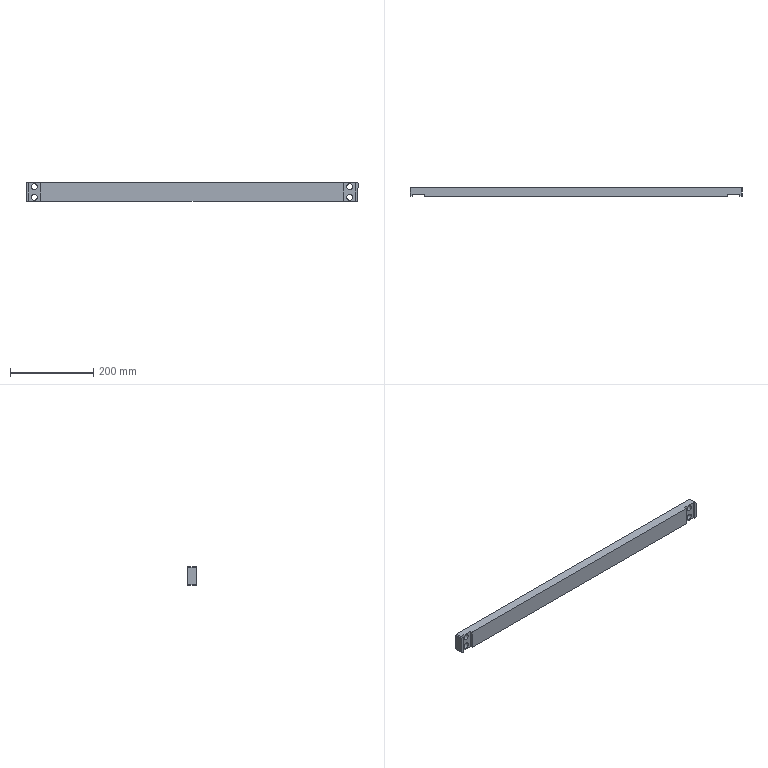Component | SolidWorks | FE5-217--p_O-1 | 1 solid | 26 faces | box 798 x 21 x 45 mm | volume 730590 mm3 | plane 18 | cylinder 8 | commonest cylinder face diameters 14 x8
build123d program:
from build123d import *

# Parameters (mm, degrees)
SKETCH1_W      = 798
SKETCH1_H      = 45
EXTRUDE1_DEPTH = 21
SKETCH2_W      = 30
SKETCH2_H      = 45
EXTRUDE2_DEPTH = 5
SKETCH3_R      = 7
EXTRUDE3_DEPTH = 401.185
CHAMFER1_SIZE  = 2


with BuildPart() as part:
    # Sketch1 → Extrude1 (new body)
    with BuildSketch(Plane(origin=(0, 0, 0), x_dir=(1, 0, 0), z_dir=(0, 1, 0))):
        Rectangle(SKETCH1_W, SKETCH1_H)
    extrude(amount=EXTRUDE1_DEPTH)

    # Sketch2 → Extrude2 (cut)
    with BuildSketch(Plane(origin=(0, 21, 0), x_dir=(1, 0, 0), z_dir=(0, 1, 0))):
        with Locations((379, 0)):
            Rectangle(SKETCH2_W, SKETCH2_H)
        with Locations((-379, 0)):
            Rectangle(SKETCH2_W, SKETCH2_H)
    extrude(amount=-EXTRUDE2_DEPTH, mode=Mode.SUBTRACT)

    # Sketch3 → Extrude3 (cut, through all)
    with BuildSketch(Plane(origin=(0, 21, 0), x_dir=(1, 0, 0), z_dir=(0, 1, 0))):
        with Locations(Location((379, 12.5, 0), (0, 0, 270))):
            Circle(SKETCH3_R)
        with Locations(Location((379, -12.5, 0), (0, 0, 270))):
            Circle(SKETCH3_R)
        with Locations(Location((-379, -12.5, 0), (0, 0, 270))):
            Circle(SKETCH3_R)
        with Locations(Location((-379, 12.5, 0), (0, 0, 270))):
            Circle(SKETCH3_R)
    extrude(amount=-EXTRUDE3_DEPTH, mode=Mode.SUBTRACT)

    # Chamfer1
    chamfer1_edges = [part.edges().sort_by_distance(p)[0] for p in [
        (-399, 10.5, -22.5),
        (399, 10.5, -22.5),
        (399, 10.5, 22.5),
        (-399, 10.5, 22.5),
    ]]
    chamfer(chamfer1_edges, length=CHAMFER1_SIZE)


solid = part.part

# Placed as in the assembly
solid = solid.moved(Location((-379, 125.5, -222.5), (180, 0, 0)))
STEP:
#1=CARTESIAN_POINT('',(-29.843,4.941,-7.992));
#2=VERTEX_POINT('',#1);
#3=CARTESIAN_POINT('',(-29.843,4.941,-8.543));
#4=VERTEX_POINT('',#3);
#5=CARTESIAN_POINT('',(-29.843,4.941,-8.268));
#6=DIRECTION('',(0.,-1.,0.));
#7=DIRECTION('',(0.,0.,1.));
#8=AXIS2_PLACEMENT_3D('',#5,#6,#7);
#9=CIRCLE('',#8,0.2756);
#10=EDGE_CURVE('',#2,#4,#9,.T.);
#11=ORIENTED_EDGE('',*,*,#10,.F.);
#12=CARTESIAN_POINT('',(-29.843,4.311,-7.992));
#13=VERTEX_POINT('',#12);
#14=CARTESIAN_POINT('',(-29.843,4.941,-7.992));
#15=DIRECTION('',(0.,-1.,0.));
#16=VECTOR('',#15,39.37);
#17=LINE('',#14,#16);
#18=EDGE_CURVE('',#2,#13,#17,.T.);
#19=ORIENTED_EDGE('',*,*,#18,.T.);
#20=CARTESIAN_POINT('',(-29.843,4.311,-8.543));
#21=VERTEX_POINT('',#20);
#22=CARTESIAN_POINT('',(-29.843,4.311,-8.268));
#23=DIRECTION('',(0.,-1.,0.));
#24=DIRECTION('',(0.,0.,-1.));
#25=AXIS2_PLACEMENT_3D('',#22,#23,#24);
#26=CIRCLE('',#25,0.2756);
#27=EDGE_CURVE('',#13,#21,#26,.T.);
#28=ORIENTED_EDGE('',*,*,#27,.T.);
#29=CARTESIAN_POINT('',(-29.843,4.941,-8.543));
#30=DIRECTION('',(0.,-1.,0.));
#31=VECTOR('',#30,39.37);
#32=LINE('',#29,#31);
#33=EDGE_CURVE('',#4,#21,#32,.T.);
#34=ORIENTED_EDGE('',*,*,#33,.F.);
#35=EDGE_LOOP('',(#11,#19,#28,#34));
#36=FACE_OUTER_BOUND('',#35,.T.);
#37=CARTESIAN_POINT('',(-29.843,4.941,-8.268));
#38=DIRECTION('',(0.,-1.,0.));
#39=DIRECTION('',(0.,0.,-1.));
#40=AXIS2_PLACEMENT_3D('',#37,#38,#39);
#41=CYLINDRICAL_SURFACE('',#40,0.2756);
#42=ADVANCED_FACE('',(#36),#41,.F.);
#43=CARTESIAN_POINT('',(-29.843,4.941,-8.976));
#44=VERTEX_POINT('',#43);
#45=CARTESIAN_POINT('',(-29.843,4.941,-9.528));
#46=VERTEX_POINT('',#45);
#47=CARTESIAN_POINT('',(-29.843,4.941,-9.252));
#48=DIRECTION('',(0.,-1.,0.));
#49=DIRECTION('',(0.,0.,-1.));
#50=AXIS2_PLACEMENT_3D('',#47,#48,#49);
#51=CIRCLE('',#50,0.2756);
#52=EDGE_CURVE('',#44,#46,#51,.T.);
#53=ORIENTED_EDGE('',*,*,#52,.F.);
#54=CARTESIAN_POINT('',(-29.843,4.311,-8.976));
#55=VERTEX_POINT('',#54);
#56=CARTESIAN_POINT('',(-29.843,4.941,-8.976));
#57=DIRECTION('',(0.,-1.,0.));
#58=VECTOR('',#57,39.37);
#59=LINE('',#56,#58);
#60=EDGE_CURVE('',#44,#55,#59,.T.);
#61=ORIENTED_EDGE('',*,*,#60,.T.);
#62=CARTESIAN_POINT('',(-29.843,4.311,-9.528));
#63=VERTEX_POINT('',#62);
#64=CARTESIAN_POINT('',(-29.843,4.311,-9.252));
#65=DIRECTION('',(0.,-1.,0.));
#66=DIRECTION('',(0.,0.,-1.));
#67=AXIS2_PLACEMENT_3D('',#64,#65,#66);
#68=CIRCLE('',#67,0.2756);
#69=EDGE_CURVE('',#55,#63,#68,.T.);
#70=ORIENTED_EDGE('',*,*,#69,.T.);
#71=CARTESIAN_POINT('',(-29.843,4.941,-9.528));
#72=DIRECTION('',(0.,-1.,0.));
#73=VECTOR('',#72,39.37);
#74=LINE('',#71,#73);
#75=EDGE_CURVE('',#46,#63,#74,.T.);
#76=ORIENTED_EDGE('',*,*,#75,.F.);
#77=EDGE_LOOP('',(#53,#61,#70,#76));
#78=FACE_OUTER_BOUND('',#77,.T.);
#79=CARTESIAN_POINT('',(-29.843,4.941,-9.252));
#80=DIRECTION('',(0.,-1.,0.));
#81=DIRECTION('',(0.,0.,-1.));
#82=AXIS2_PLACEMENT_3D('',#79,#80,#81);
#83=CYLINDRICAL_SURFACE('',#82,0.2756);
#84=ADVANCED_FACE('',(#78),#83,.F.);
#85=CARTESIAN_POINT('',(-0.,4.941,-8.976));
#86=VERTEX_POINT('',#85);
#87=CARTESIAN_POINT('',(-0.,4.941,-9.528));
#88=VERTEX_POINT('',#87);
#89=CARTESIAN_POINT('',(-0.,4.941,-9.252));
#90=DIRECTION('',(0.,-1.,0.));
#91=DIRECTION('',(0.,0.,1.));
#92=AXIS2_PLACEMENT_3D('',#89,#90,#91);
#93=CIRCLE('',#92,0.2756);
#94=EDGE_CURVE('',#86,#88,#93,.T.);
#95=ORIENTED_EDGE('',*,*,#94,.F.);
#96=CARTESIAN_POINT('',(-0.,4.311,-8.976));
#97=VERTEX_POINT('',#96);
#98=CARTESIAN_POINT('',(-0.,4.941,-8.976));
#99=DIRECTION('',(0.,-1.,0.));
#100=VECTOR('',#99,39.37);
#101=LINE('',#98,#100);
#102=EDGE_CURVE('',#86,#97,#101,.T.);
#103=ORIENTED_EDGE('',*,*,#102,.T.);
#104=CARTESIAN_POINT('',(-0.,4.311,-9.528));
#105=VERTEX_POINT('',#104);
#106=CARTESIAN_POINT('',(-0.,4.311,-9.252));
#107=DIRECTION('',(0.,-1.,0.));
#108=DIRECTION('',(-0.,0.,-1.));
#109=AXIS2_PLACEMENT_3D('',#106,#107,#108);
#110=CIRCLE('',#109,0.2756);
#111=EDGE_CURVE('',#97,#105,#110,.T.);
#112=ORIENTED_EDGE('',*,*,#111,.T.);
#113=CARTESIAN_POINT('',(-0.,4.941,-9.528));
#114=DIRECTION('',(0.,-1.,0.));
#115=VECTOR('',#114,39.37);
#116=LINE('',#113,#115);
#117=EDGE_CURVE('',#88,#105,#116,.T.);
#118=ORIENTED_EDGE('',*,*,#117,.F.);
#119=EDGE_LOOP('',(#95,#103,#112,#118));
#120=FACE_OUTER_BOUND('',#119,.T.);
#121=CARTESIAN_POINT('',(-0.,4.941,-9.252));
#122=DIRECTION('',(0.,-1.,0.));
#123=DIRECTION('',(-0.,0.,-1.));
#124=AXIS2_PLACEMENT_3D('',#121,#122,#123);
#125=CYLINDRICAL_SURFACE('',#124,0.2756);
#126=ADVANCED_FACE('',(#120),#125,.F.);
#127=CARTESIAN_POINT('',(-0.,4.941,-7.992));
#128=VERTEX_POINT('',#127);
#129=CARTESIAN_POINT('',(-0.,4.941,-8.543));
#130=VERTEX_POINT('',#129);
#131=CARTESIAN_POINT('',(-0.,4.941,-8.268));
#132=DIRECTION('',(0.,-1.,0.));
#133=DIRECTION('',(-0.,0.,-1.));
#134=AXIS2_PLACEMENT_3D('',#131,#132,#133);
#135=CIRCLE('',#134,0.2756);
#136=EDGE_CURVE('',#128,#130,#135,.T.);
#137=ORIENTED_EDGE('',*,*,#136,.F.);
#138=CARTESIAN_POINT('',(-0.,4.311,-7.992));
#139=VERTEX_POINT('',#138);
#140=CARTESIAN_POINT('',(-0.,4.941,-7.992));
#141=DIRECTION('',(0.,-1.,0.));
#142=VECTOR('',#141,39.37);
#143=LINE('',#140,#142);
#144=EDGE_CURVE('',#128,#139,#143,.T.);
#145=ORIENTED_EDGE('',*,*,#144,.T.);
#146=CARTESIAN_POINT('',(-0.,4.311,-8.543));
#147=VERTEX_POINT('',#146);
#148=CARTESIAN_POINT('',(-0.,4.311,-8.268));
#149=DIRECTION('',(0.,-1.,0.));
#150=DIRECTION('',(-0.,0.,-1.));
#151=AXIS2_PLACEMENT_3D('',#148,#149,#150);
#152=CIRCLE('',#151,0.2756);
#153=EDGE_CURVE('',#139,#147,#152,.T.);
#154=ORIENTED_EDGE('',*,*,#153,.T.);
#155=CARTESIAN_POINT('',(-0.,4.941,-8.543));
#156=DIRECTION('',(0.,-1.,0.));
#157=VECTOR('',#156,39.37);
#158=LINE('',#155,#157);
#159=EDGE_CURVE('',#130,#147,#158,.T.);
#160=ORIENTED_EDGE('',*,*,#159,.F.);
#161=EDGE_LOOP('',(#137,#145,#154,#160));
#162=FACE_OUTER_BOUND('',#161,.T.);
#163=CARTESIAN_POINT('',(-0.,4.941,-8.268));
#164=DIRECTION('',(0.,-1.,0.));
#165=DIRECTION('',(-0.,0.,-1.));
#166=AXIS2_PLACEMENT_3D('',#163,#164,#165);
#167=CYLINDRICAL_SURFACE('',#166,0.2756);
#168=ADVANCED_FACE('',(#162),#167,.F.);
#169=CARTESIAN_POINT('',(-29.252,4.114,-9.646));
#170=VERTEX_POINT('',#169);
#171=CARTESIAN_POINT('',(-29.252,4.114,-7.874));
#172=VERTEX_POINT('',#171);
#173=CARTESIAN_POINT('',(-29.252,4.114,-7.874));
#174=DIRECTION('',(0.,0.,1.));
#175=VECTOR('',#174,39.37);
#176=LINE('',#173,#175);
#177=EDGE_CURVE('',#170,#172,#176,.T.);
#178=ORIENTED_EDGE('',*,*,#177,.F.);
#179=CARTESIAN_POINT('',(-0.5906,4.114,-9.646));
#180=VERTEX_POINT('',#179);
#181=CARTESIAN_POINT('',(0.7874,4.114,-9.646));
#182=DIRECTION('',(1.,0.,-0.));
#183=VECTOR('',#182,39.37);
#184=LINE('',#181,#183);
#185=EDGE_CURVE('',#170,#180,#184,.T.);
#186=ORIENTED_EDGE('',*,*,#185,.T.);
#187=CARTESIAN_POINT('',(-0.5906,4.114,-7.874));
#188=VERTEX_POINT('',#187);
#189=CARTESIAN_POINT('',(-0.5906,4.114,-7.874));
#190=DIRECTION('',(-0.,0.,-1.));
#191=VECTOR('',#190,39.37);
#192=LINE('',#189,#191);
#193=EDGE_CURVE('',#188,#180,#192,.T.);
#194=ORIENTED_EDGE('',*,*,#193,.F.);
#195=CARTESIAN_POINT('',(0.7874,4.114,-7.874));
#196=DIRECTION('',(-1.,0.,0.));
#197=VECTOR('',#196,39.37);
#198=LINE('',#195,#197);
#199=EDGE_CURVE('',#188,#172,#198,.T.);
#200=ORIENTED_EDGE('',*,*,#199,.T.);
#201=EDGE_LOOP('',(#178,#186,#194,#200));
#202=FACE_OUTER_BOUND('',#201,.T.);
#203=CARTESIAN_POINT('',(-30.63,4.114,-7.874));
#204=DIRECTION('',(0.,-1.,0.));
#205=DIRECTION('',(-0.,0.,-1.));
#206=AXIS2_PLACEMENT_3D('',#203,#204,#205);
#207=PLANE('',#206);
#208=ADVANCED_FACE('',(#202),#207,.T.);
#209=CARTESIAN_POINT('',(-30.433,4.114,-7.874));
#210=VERTEX_POINT('',#209);
#211=CARTESIAN_POINT('',(-30.551,4.114,-7.874));
#212=VERTEX_POINT('',#211);
#213=CARTESIAN_POINT('',(0.7874,4.114,-7.874));
#214=DIRECTION('',(-1.,0.,0.));
#215=VECTOR('',#214,39.37);
#216=LINE('',#213,#215);
#217=EDGE_CURVE('',#210,#212,#216,.T.);
#218=ORIENTED_EDGE('',*,*,#217,.T.);
#219=CARTESIAN_POINT('',(-30.63,4.114,-7.953));
#220=VERTEX_POINT('',#219);
#221=CARTESIAN_POINT('',(-30.591,4.114,-7.913));
#222=DIRECTION('',(-0.7071,0.,-0.7071));
#223=VECTOR('',#222,39.37);
#224=LINE('',#221,#223);
#225=EDGE_CURVE('',#212,#220,#224,.T.);
#226=ORIENTED_EDGE('',*,*,#225,.T.);
#227=CARTESIAN_POINT('',(-30.63,4.114,-9.567));
#228=VERTEX_POINT('',#227);
#229=CARTESIAN_POINT('',(-30.63,4.114,-9.646));
#230=DIRECTION('',(-0.,0.,-1.));
#231=VECTOR('',#230,39.37);
#232=LINE('',#229,#231);
#233=EDGE_CURVE('',#220,#228,#232,.T.);
#234=ORIENTED_EDGE('',*,*,#233,.T.);
#235=CARTESIAN_POINT('',(-30.551,4.114,-9.646));
#236=VERTEX_POINT('',#235);
#237=CARTESIAN_POINT('',(-31.476,4.114,-8.72));
#238=DIRECTION('',(0.7071,0.,-0.7071));
#239=VECTOR('',#238,39.37);
#240=LINE('',#237,#239);
#241=EDGE_CURVE('',#228,#236,#240,.T.);
#242=ORIENTED_EDGE('',*,*,#241,.T.);
#243=CARTESIAN_POINT('',(-30.433,4.114,-9.646));
#244=VERTEX_POINT('',#243);
#245=CARTESIAN_POINT('',(0.7874,4.114,-9.646));
#246=DIRECTION('',(1.,0.,-0.));
#247=VECTOR('',#246,39.37);
#248=LINE('',#245,#247);
#249=EDGE_CURVE('',#236,#244,#248,.T.);
#250=ORIENTED_EDGE('',*,*,#249,.T.);
#251=CARTESIAN_POINT('',(-30.433,4.114,-7.874));
#252=DIRECTION('',(-0.,0.,-1.));
#253=VECTOR('',#252,39.37);
#254=LINE('',#251,#253);
#255=EDGE_CURVE('',#210,#244,#254,.T.);
#256=ORIENTED_EDGE('',*,*,#255,.F.);
#257=EDGE_LOOP('',(#218,#226,#234,#242,#250,#256));
#258=FACE_OUTER_BOUND('',#257,.T.);
#259=CARTESIAN_POINT('',(-30.63,4.114,-7.874));
#260=DIRECTION('',(0.,-1.,0.));
#261=DIRECTION('',(-0.,0.,-1.));
#262=AXIS2_PLACEMENT_3D('',#259,#260,#261);
#263=PLANE('',#262);
#264=ADVANCED_FACE('',(#258),#263,.T.);
#265=ORIENTED_EDGE('',*,*,#233,.F.);
#266=CARTESIAN_POINT('',(-30.63,4.941,-7.953));
#267=VERTEX_POINT('',#266);
#268=CARTESIAN_POINT('',(-30.63,4.114,-7.953));
#269=DIRECTION('',(0.,1.,0.));
#270=VECTOR('',#269,39.37);
#271=LINE('',#268,#270);
#272=EDGE_CURVE('',#220,#267,#271,.T.);
#273=ORIENTED_EDGE('',*,*,#272,.T.);
#274=CARTESIAN_POINT('',(-30.63,4.941,-9.567));
#275=VERTEX_POINT('',#274);
#276=CARTESIAN_POINT('',(-30.63,4.941,-9.646));
#277=DIRECTION('',(-0.,0.,-1.));
#278=VECTOR('',#277,39.37);
#279=LINE('',#276,#278);
#280=EDGE_CURVE('',#267,#275,#279,.T.);
#281=ORIENTED_EDGE('',*,*,#280,.T.);
#282=CARTESIAN_POINT('',(-30.63,4.114,-9.567));
#283=DIRECTION('',(0.,-1.,0.));
#284=VECTOR('',#283,39.37);
#285=LINE('',#282,#284);
#286=EDGE_CURVE('',#275,#228,#285,.T.);
#287=ORIENTED_EDGE('',*,*,#286,.T.);
#288=EDGE_LOOP('',(#265,#273,#281,#287));
#289=FACE_OUTER_BOUND('',#288,.T.);
#290=CARTESIAN_POINT('',(-30.63,4.114,-9.646));
#291=DIRECTION('',(1.,0.,-0.));
#292=DIRECTION('',(0.,0.,1.));
#293=AXIS2_PLACEMENT_3D('',#290,#291,#292);
#294=PLANE('',#293);
#295=ADVANCED_FACE('',(#289),#294,.F.);
#296=ORIENTED_EDGE('',*,*,#249,.F.);
#297=CARTESIAN_POINT('',(-30.551,4.941,-9.646));
#298=VERTEX_POINT('',#297);
#299=CARTESIAN_POINT('',(-30.551,4.114,-9.646));
#300=DIRECTION('',(0.,1.,0.));
#301=VECTOR('',#300,39.37);
#302=LINE('',#299,#301);
#303=EDGE_CURVE('',#236,#298,#302,.T.);
#304=ORIENTED_EDGE('',*,*,#303,.T.);
#305=CARTESIAN_POINT('',(0.7087,4.941,-9.646));
#306=VERTEX_POINT('',#305);
#307=CARTESIAN_POINT('',(0.7874,4.941,-9.646));
#308=DIRECTION('',(1.,0.,-0.));
#309=VECTOR('',#308,39.37);
#310=LINE('',#307,#309);
#311=EDGE_CURVE('',#298,#306,#310,.T.);
#312=ORIENTED_EDGE('',*,*,#311,.T.);
#313=CARTESIAN_POINT('',(0.7087,4.114,-9.646));
#314=VERTEX_POINT('',#313);
#315=CARTESIAN_POINT('',(0.7087,4.114,-9.646));
#316=DIRECTION('',(0.,-1.,0.));
#317=VECTOR('',#316,39.37);
#318=LINE('',#315,#317);
#319=EDGE_CURVE('',#306,#314,#318,.T.);
#320=ORIENTED_EDGE('',*,*,#319,.T.);
#321=CARTESIAN_POINT('',(0.5906,4.114,-9.646));
#322=VERTEX_POINT('',#321);
#323=CARTESIAN_POINT('',(0.7874,4.114,-9.646));
#324=DIRECTION('',(1.,0.,-0.));
#325=VECTOR('',#324,39.37);
#326=LINE('',#323,#325);
#327=EDGE_CURVE('',#322,#314,#326,.T.);
#328=ORIENTED_EDGE('',*,*,#327,.F.);
#329=CARTESIAN_POINT('',(0.5906,4.311,-9.646));
#330=VERTEX_POINT('',#329);
#331=CARTESIAN_POINT('',(0.5906,4.311,-9.646));
#332=DIRECTION('',(0.,-1.,0.));
#333=VECTOR('',#332,39.37);
#334=LINE('',#331,#333);
#335=EDGE_CURVE('',#330,#322,#334,.T.);
#336=ORIENTED_EDGE('',*,*,#335,.F.);
#337=CARTESIAN_POINT('',(-0.5906,4.311,-9.646));
#338=VERTEX_POINT('',#337);
#339=CARTESIAN_POINT('',(-0.5906,4.311,-9.646));
#340=DIRECTION('',(1.,0.,-0.));
#341=VECTOR('',#340,39.37);
#342=LINE('',#339,#341);
#343=EDGE_CURVE('',#338,#330,#342,.T.);
#344=ORIENTED_EDGE('',*,*,#343,.F.);
#345=CARTESIAN_POINT('',(-0.5906,4.311,-9.646));
#346=DIRECTION('',(0.,-1.,0.));
#347=VECTOR('',#346,39.37);
#348=LINE('',#345,#347);
#349=EDGE_CURVE('',#338,#180,#348,.T.);
#350=ORIENTED_EDGE('',*,*,#349,.T.);
#351=ORIENTED_EDGE('',*,*,#185,.F.);
#352=CARTESIAN_POINT('',(-29.252,4.311,-9.646));
#353=VERTEX_POINT('',#352);
#354=CARTESIAN_POINT('',(-29.252,4.311,-9.646));
#355=DIRECTION('',(0.,-1.,0.));
#356=VECTOR('',#355,39.37);
#357=LINE('',#354,#356);
#358=EDGE_CURVE('',#353,#170,#357,.T.);
#359=ORIENTED_EDGE('',*,*,#358,.F.);
#360=CARTESIAN_POINT('',(-30.433,4.311,-9.646));
#361=VERTEX_POINT('',#360);
#362=CARTESIAN_POINT('',(-29.252,4.311,-9.646));
#363=DIRECTION('',(1.,0.,-0.));
#364=VECTOR('',#363,39.37);
#365=LINE('',#362,#364);
#366=EDGE_CURVE('',#361,#353,#365,.T.);
#367=ORIENTED_EDGE('',*,*,#366,.F.);
#368=CARTESIAN_POINT('',(-30.433,4.311,-9.646));
#369=DIRECTION('',(0.,-1.,0.));
#370=VECTOR('',#369,39.37);
#371=LINE('',#368,#370);
#372=EDGE_CURVE('',#361,#244,#371,.T.);
#373=ORIENTED_EDGE('',*,*,#372,.T.);
#374=EDGE_LOOP('',(#296,#304,#312,#320,#328,#336,#344,#350,#351,#359,#367,#373));
#375=FACE_OUTER_BOUND('',#374,.T.);
#376=CARTESIAN_POINT('',(0.7874,4.114,-9.646));
#377=DIRECTION('',(0.,0.,1.));
#378=DIRECTION('',(-1.,0.,0.));
#379=AXIS2_PLACEMENT_3D('',#376,#377,#378);
#380=PLANE('',#379);
#381=ADVANCED_FACE('',(#375),#380,.F.);
#382=CARTESIAN_POINT('',(0.7874,4.941,-9.567));
#383=VERTEX_POINT('',#382);
#384=CARTESIAN_POINT('',(0.7874,4.941,-7.953));
#385=VERTEX_POINT('',#384);
#386=CARTESIAN_POINT('',(0.7874,4.941,-9.646));
#387=DIRECTION('',(0.,0.,1.));
#388=VECTOR('',#387,39.37);
#389=LINE('',#386,#388);
#390=EDGE_CURVE('',#383,#385,#389,.T.);
#391=ORIENTED_EDGE('',*,*,#390,.T.);
#392=CARTESIAN_POINT('',(0.7874,4.114,-7.953));
#393=VERTEX_POINT('',#392);
#394=CARTESIAN_POINT('',(0.7874,4.114,-7.953));
#395=DIRECTION('',(0.,-1.,0.));
#396=VECTOR('',#395,39.37);
#397=LINE('',#394,#396);
#398=EDGE_CURVE('',#385,#393,#397,.T.);
#399=ORIENTED_EDGE('',*,*,#398,.T.);
#400=CARTESIAN_POINT('',(0.7874,4.114,-9.567));
#401=VERTEX_POINT('',#400);
#402=CARTESIAN_POINT('',(0.7874,4.114,-9.646));
#403=DIRECTION('',(0.,0.,1.));
#404=VECTOR('',#403,39.37);
#405=LINE('',#402,#404);
#406=EDGE_CURVE('',#401,#393,#405,.T.);
#407=ORIENTED_EDGE('',*,*,#406,.F.);
#408=CARTESIAN_POINT('',(0.7874,4.114,-9.567));
#409=DIRECTION('',(0.,1.,0.));
#410=VECTOR('',#409,39.37);
#411=LINE('',#408,#410);
#412=EDGE_CURVE('',#401,#383,#411,.T.);
#413=ORIENTED_EDGE('',*,*,#412,.T.);
#414=EDGE_LOOP('',(#391,#399,#407,#413));
#415=FACE_OUTER_BOUND('',#414,.T.);
#416=CARTESIAN_POINT('',(0.7874,4.114,-9.646));
#417=DIRECTION('',(-1.,0.,0.));
#418=DIRECTION('',(-0.,0.,-1.));
#419=AXIS2_PLACEMENT_3D('',#416,#417,#418);
#420=PLANE('',#419);
#421=ADVANCED_FACE('',(#415),#420,.F.);
#422=CARTESIAN_POINT('',(0.7087,4.941,-7.874));
#423=VERTEX_POINT('',#422);
#424=CARTESIAN_POINT('',(-30.551,4.941,-7.874));
#425=VERTEX_POINT('',#424);
#426=CARTESIAN_POINT('',(0.7874,4.941,-7.874));
#427=DIRECTION('',(-1.,0.,0.));
#428=VECTOR('',#427,39.37);
#429=LINE('',#426,#428);
#430=EDGE_CURVE('',#423,#425,#429,.T.);
#431=ORIENTED_EDGE('',*,*,#430,.T.);
#432=CARTESIAN_POINT('',(-30.551,4.114,-7.874));
#433=DIRECTION('',(0.,-1.,0.));
#434=VECTOR('',#433,39.37);
#435=LINE('',#432,#434);
#436=EDGE_CURVE('',#425,#212,#435,.T.);
#437=ORIENTED_EDGE('',*,*,#436,.T.);
#438=ORIENTED_EDGE('',*,*,#217,.F.);
#439=CARTESIAN_POINT('',(-30.433,4.311,-7.874));
#440=VERTEX_POINT('',#439);
#441=CARTESIAN_POINT('',(-30.433,4.311,-7.874));
#442=DIRECTION('',(0.,-1.,0.));
#443=VECTOR('',#442,39.37);
#444=LINE('',#441,#443);
#445=EDGE_CURVE('',#440,#210,#444,.T.);
#446=ORIENTED_EDGE('',*,*,#445,.F.);
#447=CARTESIAN_POINT('',(-29.252,4.311,-7.874));
#448=VERTEX_POINT('',#447);
#449=CARTESIAN_POINT('',(-29.252,4.311,-7.874));
#450=DIRECTION('',(-1.,0.,0.));
#451=VECTOR('',#450,39.37);
#452=LINE('',#449,#451);
#453=EDGE_CURVE('',#448,#440,#452,.T.);
#454=ORIENTED_EDGE('',*,*,#453,.F.);
#455=CARTESIAN_POINT('',(-29.252,4.311,-7.874));
#456=DIRECTION('',(0.,-1.,0.));
#457=VECTOR('',#456,39.37);
#458=LINE('',#455,#457);
#459=EDGE_CURVE('',#448,#172,#458,.T.);
#460=ORIENTED_EDGE('',*,*,#459,.T.);
#461=ORIENTED_EDGE('',*,*,#199,.F.);
#462=CARTESIAN_POINT('',(-0.5906,4.311,-7.874));
#463=VERTEX_POINT('',#462);
#464=CARTESIAN_POINT('',(-0.5906,4.311,-7.874));
#465=DIRECTION('',(0.,-1.,0.));
#466=VECTOR('',#465,39.37);
#467=LINE('',#464,#466);
#468=EDGE_CURVE('',#463,#188,#467,.T.);
#469=ORIENTED_EDGE('',*,*,#468,.F.);
#470=CARTESIAN_POINT('',(0.5906,4.311,-7.874));
#471=VERTEX_POINT('',#470);
#472=CARTESIAN_POINT('',(-0.5906,4.311,-7.874));
#473=DIRECTION('',(-1.,0.,0.));
#474=VECTOR('',#473,39.37);
#475=LINE('',#472,#474);
#476=EDGE_CURVE('',#471,#463,#475,.T.);
#477=ORIENTED_EDGE('',*,*,#476,.F.);
#478=CARTESIAN_POINT('',(0.5906,4.114,-7.874));
#479=VERTEX_POINT('',#478);
#480=CARTESIAN_POINT('',(0.5906,4.311,-7.874));
#481=DIRECTION('',(0.,-1.,0.));
#482=VECTOR('',#481,39.37);
#483=LINE('',#480,#482);
#484=EDGE_CURVE('',#471,#479,#483,.T.);
#485=ORIENTED_EDGE('',*,*,#484,.T.);
#486=CARTESIAN_POINT('',(0.7087,4.114,-7.874));
#487=VERTEX_POINT('',#486);
#488=CARTESIAN_POINT('',(0.7874,4.114,-7.874));
#489=DIRECTION('',(-1.,0.,0.));
#490=VECTOR('',#489,39.37);
#491=LINE('',#488,#490);
#492=EDGE_CURVE('',#487,#479,#491,.T.);
#493=ORIENTED_EDGE('',*,*,#492,.F.);
#494=CARTESIAN_POINT('',(0.7087,4.114,-7.874));
#495=DIRECTION('',(0.,1.,0.));
#496=VECTOR('',#495,39.37);
#497=LINE('',#494,#496);
#498=EDGE_CURVE('',#487,#423,#497,.T.);
#499=ORIENTED_EDGE('',*,*,#498,.T.);
#500=EDGE_LOOP('',(#431,#437,#438,#446,#454,#460,#461,#469,#477,#485,#493,#499));
#501=FACE_OUTER_BOUND('',#500,.T.);
#502=CARTESIAN_POINT('',(0.7874,4.114,-7.874));
#503=DIRECTION('',(-0.,0.,-1.));
#504=DIRECTION('',(1.,0.,-0.));
#505=AXIS2_PLACEMENT_3D('',#502,#503,#504);
#506=PLANE('',#505);
#507=ADVANCED_FACE('',(#501),#506,.F.);
#508=ORIENTED_EDGE('',*,*,#406,.T.);
#509=CARTESIAN_POINT('',(-14.961,4.114,7.795));
#510=DIRECTION('',(-0.7071,0.,0.7071));
#511=VECTOR('',#510,39.37);
#512=LINE('',#509,#511);
#513=EDGE_CURVE('',#393,#487,#512,.T.);
#514=ORIENTED_EDGE('',*,*,#513,.T.);
#515=ORIENTED_EDGE('',*,*,#492,.T.);
#516=CARTESIAN_POINT('',(0.5906,4.114,-7.874));
#517=DIRECTION('',(0.,0.,1.));
#518=VECTOR('',#517,39.37);
#519=LINE('',#516,#518);
#520=EDGE_CURVE('',#322,#479,#519,.T.);
#521=ORIENTED_EDGE('',*,*,#520,.F.);
#522=ORIENTED_EDGE('',*,*,#327,.T.);
#523=CARTESIAN_POINT('',(-14.075,4.114,-24.429));
#524=DIRECTION('',(0.7071,0.,0.7071));
#525=VECTOR('',#524,39.37);
#526=LINE('',#523,#525);
#527=EDGE_CURVE('',#314,#401,#526,.T.);
#528=ORIENTED_EDGE('',*,*,#527,.T.);
#529=EDGE_LOOP('',(#508,#514,#515,#521,#522,#528));
#530=FACE_OUTER_BOUND('',#529,.T.);
#531=CARTESIAN_POINT('',(-30.63,4.114,-7.874));
#532=DIRECTION('',(0.,-1.,0.));
#533=DIRECTION('',(-0.,0.,-1.));
#534=AXIS2_PLACEMENT_3D('',#531,#532,#533);
#535=PLANE('',#534);
#536=ADVANCED_FACE('',(#530),#535,.T.);
#537=CARTESIAN_POINT('',(-29.843,4.941,-8.268));
#538=DIRECTION('',(0.,-1.,0.));
#539=DIRECTION('',(0.,0.,1.));
#540=AXIS2_PLACEMENT_3D('',#537,#538,#539);
#541=CIRCLE('',#540,0.2756);
#542=EDGE_CURVE('',#4,#2,#541,.T.);
#543=ORIENTED_EDGE('',*,*,#542,.T.);
#544=ORIENTED_EDGE('',*,*,#10,.T.);
#545=EDGE_LOOP('',(#543,#544));
#546=FACE_BOUND('',#545,.T.);
#547=CARTESIAN_POINT('',(-29.843,4.941,-9.252));
#548=DIRECTION('',(0.,-1.,0.));
#549=DIRECTION('',(0.,0.,-1.));
#550=AXIS2_PLACEMENT_3D('',#547,#548,#549);
#551=CIRCLE('',#550,0.2756);
#552=EDGE_CURVE('',#46,#44,#551,.T.);
#553=ORIENTED_EDGE('',*,*,#552,.T.);
#554=ORIENTED_EDGE('',*,*,#52,.T.);
#555=EDGE_LOOP('',(#553,#554));
#556=FACE_BOUND('',#555,.T.);
#557=CARTESIAN_POINT('',(-0.,4.941,-9.252));
#558=DIRECTION('',(0.,-1.,0.));
#559=DIRECTION('',(0.,0.,1.));
#560=AXIS2_PLACEMENT_3D('',#557,#558,#559);
#561=CIRCLE('',#560,0.2756);
#562=EDGE_CURVE('',#88,#86,#561,.T.);
#563=ORIENTED_EDGE('',*,*,#562,.T.);
#564=ORIENTED_EDGE('',*,*,#94,.T.);
#565=EDGE_LOOP('',(#563,#564));
#566=FACE_BOUND('',#565,.T.);
#567=CARTESIAN_POINT('',(-0.,4.941,-8.268));
#568=DIRECTION('',(0.,-1.,0.));
#569=DIRECTION('',(-0.,0.,-1.));
#570=AXIS2_PLACEMENT_3D('',#567,#568,#569);
#571=CIRCLE('',#570,0.2756);
#572=EDGE_CURVE('',#130,#128,#571,.T.);
#573=ORIENTED_EDGE('',*,*,#572,.T.);
#574=ORIENTED_EDGE('',*,*,#136,.T.);
#575=EDGE_LOOP('',(#573,#574));
#576=FACE_BOUND('',#575,.T.);
#577=ORIENTED_EDGE('',*,*,#280,.F.);
#578=CARTESIAN_POINT('',(-30.63,4.941,-7.953));
#579=DIRECTION('',(0.7071,0.,0.7071));
#580=VECTOR('',#579,39.37);
#581=LINE('',#578,#580);
#582=EDGE_CURVE('',#267,#425,#581,.T.);
#583=ORIENTED_EDGE('',*,*,#582,.T.);
#584=ORIENTED_EDGE('',*,*,#430,.F.);
#585=CARTESIAN_POINT('',(0.7087,4.941,-7.874));
#586=DIRECTION('',(0.7071,0.,-0.7071));
#587=VECTOR('',#586,39.37);
#588=LINE('',#585,#587);
#589=EDGE_CURVE('',#423,#385,#588,.T.);
#590=ORIENTED_EDGE('',*,*,#589,.T.);
#591=ORIENTED_EDGE('',*,*,#390,.F.);
#592=CARTESIAN_POINT('',(0.7874,4.941,-9.567));
#593=DIRECTION('',(-0.7071,0.,-0.7071));
#594=VECTOR('',#593,39.37);
#595=LINE('',#592,#594);
#596=EDGE_CURVE('',#383,#306,#595,.T.);
#597=ORIENTED_EDGE('',*,*,#596,.T.);
#598=ORIENTED_EDGE('',*,*,#311,.F.);
#599=CARTESIAN_POINT('',(-30.551,4.941,-9.646));
#600=DIRECTION('',(-0.7071,0.,0.7071));
#601=VECTOR('',#600,39.37);
#602=LINE('',#599,#601);
#603=EDGE_CURVE('',#298,#275,#602,.T.);
#604=ORIENTED_EDGE('',*,*,#603,.T.);
#605=EDGE_LOOP('',(#577,#583,#584,#590,#591,#597,#598,#604));
#606=FACE_OUTER_BOUND('',#605,.T.);
#607=CARTESIAN_POINT('',(-30.63,4.941,-7.874));
#608=DIRECTION('',(0.,-1.,0.));
#609=DIRECTION('',(-0.,0.,-1.));
#610=AXIS2_PLACEMENT_3D('',#607,#608,#609);
#611=PLANE('',#610);
#612=ADVANCED_FACE('',(#546,#556,#566,#576,#606),#611,.F.);
#613=ORIENTED_EDGE('',*,*,#193,.T.);
#614=ORIENTED_EDGE('',*,*,#349,.F.);
#615=CARTESIAN_POINT('',(-0.5906,4.311,-7.874));
#616=DIRECTION('',(-0.,0.,-1.));
#617=VECTOR('',#616,39.37);
#618=LINE('',#615,#617);
#619=EDGE_CURVE('',#463,#338,#618,.T.);
#620=ORIENTED_EDGE('',*,*,#619,.F.);
#621=ORIENTED_EDGE('',*,*,#468,.T.);
#622=EDGE_LOOP('',(#613,#614,#620,#621));
#623=FACE_OUTER_BOUND('',#622,.T.);
#624=CARTESIAN_POINT('',(-0.5906,4.311,-7.874));
#625=DIRECTION('',(-1.,0.,0.));
#626=DIRECTION('',(-0.,0.,-1.));
#627=AXIS2_PLACEMENT_3D('',#624,#625,#626);
#628=PLANE('',#627);
#629=ADVANCED_FACE('',(#623),#628,.F.);
#630=ORIENTED_EDGE('',*,*,#520,.T.);
#631=ORIENTED_EDGE('',*,*,#484,.F.);
#632=CARTESIAN_POINT('',(0.5906,4.311,-7.874));
#633=DIRECTION('',(0.,0.,1.));
#634=VECTOR('',#633,39.37);
#635=LINE('',#632,#634);
#636=EDGE_CURVE('',#330,#471,#635,.T.);
#637=ORIENTED_EDGE('',*,*,#636,.F.);
#638=ORIENTED_EDGE('',*,*,#335,.T.);
#639=EDGE_LOOP('',(#630,#631,#637,#638));
#640=FACE_OUTER_BOUND('',#639,.T.);
#641=CARTESIAN_POINT('',(0.5906,4.311,-7.874));
#642=DIRECTION('',(1.,0.,-0.));
#643=DIRECTION('',(0.,0.,1.));
#644=AXIS2_PLACEMENT_3D('',#641,#642,#643);
#645=PLANE('',#644);
#646=ADVANCED_FACE('',(#640),#645,.F.);
#647=CARTESIAN_POINT('',(-0.,4.311,-9.252));
#648=DIRECTION('',(0.,-1.,0.));
#649=DIRECTION('',(-0.,0.,-1.));
#650=AXIS2_PLACEMENT_3D('',#647,#648,#649);
#651=CIRCLE('',#650,0.2756);
#652=EDGE_CURVE('',#105,#97,#651,.T.);
#653=ORIENTED_EDGE('',*,*,#652,.F.);
#654=ORIENTED_EDGE('',*,*,#111,.F.);
#655=EDGE_LOOP('',(#653,#654));
#656=FACE_BOUND('',#655,.T.);
#657=CARTESIAN_POINT('',(-0.,4.311,-8.268));
#658=DIRECTION('',(0.,-1.,0.));
#659=DIRECTION('',(-0.,0.,-1.));
#660=AXIS2_PLACEMENT_3D('',#657,#658,#659);
#661=CIRCLE('',#660,0.2756);
#662=EDGE_CURVE('',#147,#139,#661,.T.);
#663=ORIENTED_EDGE('',*,*,#662,.F.);
#664=ORIENTED_EDGE('',*,*,#153,.F.);
#665=EDGE_LOOP('',(#663,#664));
#666=FACE_BOUND('',#665,.T.);
#667=ORIENTED_EDGE('',*,*,#619,.T.);
#668=ORIENTED_EDGE('',*,*,#343,.T.);
#669=ORIENTED_EDGE('',*,*,#636,.T.);
#670=ORIENTED_EDGE('',*,*,#476,.T.);
#671=EDGE_LOOP('',(#667,#668,#669,#670));
#672=FACE_OUTER_BOUND('',#671,.T.);
#673=CARTESIAN_POINT('',(-0.5906,4.311,-9.646));
#674=DIRECTION('',(0.,-1.,0.));
#675=DIRECTION('',(-0.,0.,-1.));
#676=AXIS2_PLACEMENT_3D('',#673,#674,#675);
#677=PLANE('',#676);
#678=ADVANCED_FACE('',(#656,#666,#672),#677,.T.);
#679=ORIENTED_EDGE('',*,*,#177,.T.);
#680=ORIENTED_EDGE('',*,*,#459,.F.);
#681=CARTESIAN_POINT('',(-29.252,4.311,-7.874));
#682=DIRECTION('',(0.,0.,1.));
#683=VECTOR('',#682,39.37);
#684=LINE('',#681,#683);
#685=EDGE_CURVE('',#353,#448,#684,.T.);
#686=ORIENTED_EDGE('',*,*,#685,.F.);
#687=ORIENTED_EDGE('',*,*,#358,.T.);
#688=EDGE_LOOP('',(#679,#680,#686,#687));
#689=FACE_OUTER_BOUND('',#688,.T.);
#690=CARTESIAN_POINT('',(-29.252,4.311,-7.874));
#691=DIRECTION('',(1.,0.,-0.));
#692=DIRECTION('',(0.,0.,1.));
#693=AXIS2_PLACEMENT_3D('',#690,#691,#692);
#694=PLANE('',#693);
#695=ADVANCED_FACE('',(#689),#694,.F.);
#696=ORIENTED_EDGE('',*,*,#255,.T.);
#697=ORIENTED_EDGE('',*,*,#372,.F.);
#698=CARTESIAN_POINT('',(-30.433,4.311,-7.874));
#699=DIRECTION('',(-0.,0.,-1.));
#700=VECTOR('',#699,39.37);
#701=LINE('',#698,#700);
#702=EDGE_CURVE('',#440,#361,#701,.T.);
#703=ORIENTED_EDGE('',*,*,#702,.F.);
#704=ORIENTED_EDGE('',*,*,#445,.T.);
#705=EDGE_LOOP('',(#696,#697,#703,#704));
#706=FACE_OUTER_BOUND('',#705,.T.);
#707=CARTESIAN_POINT('',(-30.433,4.311,-7.874));
#708=DIRECTION('',(-1.,0.,0.));
#709=DIRECTION('',(-0.,0.,-1.));
#710=AXIS2_PLACEMENT_3D('',#707,#708,#709);
#711=PLANE('',#710);
#712=ADVANCED_FACE('',(#706),#711,.F.);
#713=CARTESIAN_POINT('',(-29.843,4.311,-8.268));
#714=DIRECTION('',(0.,-1.,0.));
#715=DIRECTION('',(0.,0.,-1.));
#716=AXIS2_PLACEMENT_3D('',#713,#714,#715);
#717=CIRCLE('',#716,0.2756);
#718=EDGE_CURVE('',#21,#13,#717,.T.);
#719=ORIENTED_EDGE('',*,*,#718,.F.);
#720=ORIENTED_EDGE('',*,*,#27,.F.);
#721=EDGE_LOOP('',(#719,#720));
#722=FACE_BOUND('',#721,.T.);
#723=CARTESIAN_POINT('',(-29.843,4.311,-9.252));
#724=DIRECTION('',(0.,-1.,0.));
#725=DIRECTION('',(0.,0.,-1.));
#726=AXIS2_PLACEMENT_3D('',#723,#724,#725);
#727=CIRCLE('',#726,0.2756);
#728=EDGE_CURVE('',#63,#55,#727,.T.);
#729=ORIENTED_EDGE('',*,*,#728,.F.);
#730=ORIENTED_EDGE('',*,*,#69,.F.);
#731=EDGE_LOOP('',(#729,#730));
#732=FACE_BOUND('',#731,.T.);
#733=ORIENTED_EDGE('',*,*,#453,.T.);
#734=ORIENTED_EDGE('',*,*,#702,.T.);
#735=ORIENTED_EDGE('',*,*,#366,.T.);
#736=ORIENTED_EDGE('',*,*,#685,.T.);
#737=EDGE_LOOP('',(#733,#734,#735,#736));
#738=FACE_OUTER_BOUND('',#737,.T.);
#739=CARTESIAN_POINT('',(-30.433,4.311,-7.874));
#740=DIRECTION('',(0.,-1.,0.));
#741=DIRECTION('',(-0.,0.,-1.));
#742=AXIS2_PLACEMENT_3D('',#739,#740,#741);
#743=PLANE('',#742);
#744=ADVANCED_FACE('',(#722,#732,#738),#743,.T.);
#745=ORIENTED_EDGE('',*,*,#144,.F.);
#746=ORIENTED_EDGE('',*,*,#572,.F.);
#747=ORIENTED_EDGE('',*,*,#159,.T.);
#748=ORIENTED_EDGE('',*,*,#662,.T.);
#749=EDGE_LOOP('',(#745,#746,#747,#748));
#750=FACE_OUTER_BOUND('',#749,.T.);
#751=CARTESIAN_POINT('',(-0.,4.941,-8.268));
#752=DIRECTION('',(0.,-1.,0.));
#753=DIRECTION('',(-0.,0.,-1.));
#754=AXIS2_PLACEMENT_3D('',#751,#752,#753);
#755=CYLINDRICAL_SURFACE('',#754,0.2756);
#756=ADVANCED_FACE('',(#750),#755,.F.);
#757=ORIENTED_EDGE('',*,*,#102,.F.);
#758=ORIENTED_EDGE('',*,*,#562,.F.);
#759=ORIENTED_EDGE('',*,*,#117,.T.);
#760=ORIENTED_EDGE('',*,*,#652,.T.);
#761=EDGE_LOOP('',(#757,#758,#759,#760));
#762=FACE_OUTER_BOUND('',#761,.T.);
#763=CARTESIAN_POINT('',(-0.,4.941,-9.252));
#764=DIRECTION('',(0.,-1.,0.));
#765=DIRECTION('',(-0.,0.,-1.));
#766=AXIS2_PLACEMENT_3D('',#763,#764,#765);
#767=CYLINDRICAL_SURFACE('',#766,0.2756);
#768=ADVANCED_FACE('',(#762),#767,.F.);
#769=ORIENTED_EDGE('',*,*,#60,.F.);
#770=ORIENTED_EDGE('',*,*,#552,.F.);
#771=ORIENTED_EDGE('',*,*,#75,.T.);
#772=ORIENTED_EDGE('',*,*,#728,.T.);
#773=EDGE_LOOP('',(#769,#770,#771,#772));
#774=FACE_OUTER_BOUND('',#773,.T.);
#775=CARTESIAN_POINT('',(-29.843,4.941,-9.252));
#776=DIRECTION('',(0.,-1.,0.));
#777=DIRECTION('',(0.,0.,-1.));
#778=AXIS2_PLACEMENT_3D('',#775,#776,#777);
#779=CYLINDRICAL_SURFACE('',#778,0.2756);
#780=ADVANCED_FACE('',(#774),#779,.F.);
#781=ORIENTED_EDGE('',*,*,#18,.F.);
#782=ORIENTED_EDGE('',*,*,#542,.F.);
#783=ORIENTED_EDGE('',*,*,#33,.T.);
#784=ORIENTED_EDGE('',*,*,#718,.T.);
#785=EDGE_LOOP('',(#781,#782,#783,#784));
#786=FACE_OUTER_BOUND('',#785,.T.);
#787=CARTESIAN_POINT('',(-29.843,4.941,-8.268));
#788=DIRECTION('',(0.,-1.,0.));
#789=DIRECTION('',(0.,0.,-1.));
#790=AXIS2_PLACEMENT_3D('',#787,#788,#789);
#791=CYLINDRICAL_SURFACE('',#790,0.2756);
#792=ADVANCED_FACE('',(#786),#791,.F.);
#793=ORIENTED_EDGE('',*,*,#225,.F.);
#794=ORIENTED_EDGE('',*,*,#436,.F.);
#795=ORIENTED_EDGE('',*,*,#582,.F.);
#796=ORIENTED_EDGE('',*,*,#272,.F.);
#797=EDGE_LOOP('',(#793,#794,#795,#796));
#798=FACE_OUTER_BOUND('',#797,.T.);
#799=CARTESIAN_POINT('',(-30.63,4.114,-7.953));
#800=DIRECTION('',(0.7071,0.,-0.7071));
#801=DIRECTION('',(0.7071,0.,0.7071));
#802=AXIS2_PLACEMENT_3D('',#799,#800,#801);
#803=PLANE('',#802);
#804=ADVANCED_FACE('',(#798),#803,.F.);
#805=ORIENTED_EDGE('',*,*,#241,.F.);
#806=ORIENTED_EDGE('',*,*,#286,.F.);
#807=ORIENTED_EDGE('',*,*,#603,.F.);
#808=ORIENTED_EDGE('',*,*,#303,.F.);
#809=EDGE_LOOP('',(#805,#806,#807,#808));
#810=FACE_OUTER_BOUND('',#809,.T.);
#811=CARTESIAN_POINT('',(-30.551,4.114,-9.646));
#812=DIRECTION('',(0.7071,0.,0.7071));
#813=DIRECTION('',(-0.7071,0.,0.7071));
#814=AXIS2_PLACEMENT_3D('',#811,#812,#813);
#815=PLANE('',#814);
#816=ADVANCED_FACE('',(#810),#815,.F.);
#817=ORIENTED_EDGE('',*,*,#513,.F.);
#818=ORIENTED_EDGE('',*,*,#398,.F.);
#819=ORIENTED_EDGE('',*,*,#589,.F.);
#820=ORIENTED_EDGE('',*,*,#498,.F.);
#821=EDGE_LOOP('',(#817,#818,#819,#820));
#822=FACE_OUTER_BOUND('',#821,.T.);
#823=CARTESIAN_POINT('',(0.7087,4.114,-7.874));
#824=DIRECTION('',(-0.7071,0.,-0.7071));
#825=DIRECTION('',(0.7071,0.,-0.7071));
#826=AXIS2_PLACEMENT_3D('',#823,#824,#825);
#827=PLANE('',#826);
#828=ADVANCED_FACE('',(#822),#827,.F.);
#829=ORIENTED_EDGE('',*,*,#527,.F.);
#830=ORIENTED_EDGE('',*,*,#319,.F.);
#831=ORIENTED_EDGE('',*,*,#596,.F.);
#832=ORIENTED_EDGE('',*,*,#412,.F.);
#833=EDGE_LOOP('',(#829,#830,#831,#832));
#834=FACE_OUTER_BOUND('',#833,.T.);
#835=CARTESIAN_POINT('',(0.7874,4.114,-9.567));
#836=DIRECTION('',(-0.7071,0.,0.7071));
#837=DIRECTION('',(-0.7071,0.,-0.7071));
#838=AXIS2_PLACEMENT_3D('',#835,#836,#837);
#839=PLANE('',#838);
#840=ADVANCED_FACE('',(#834),#839,.F.);
#841=CLOSED_SHELL('',(#42,#84,#126,#168,#208,#264,#295,#381,#421,#507,#536,#612,#629,#646,#678,#695,#712,#744,#756,#768,#780,#792,#804,#816,#828,#840));
#842=MANIFOLD_SOLID_BREP('',#841);
#843=CARTESIAN_POINT('',(0.,0.,0.));
#844=DIRECTION('',(0.,0.,1.));
#845=DIRECTION('',(1.,0.,0.));
#846=AXIS2_PLACEMENT_3D('',#843,#844,#845);
#847=(LENGTH_UNIT()NAMED_UNIT(*)SI_UNIT($,.METRE.));
#848=LENGTH_MEASURE_WITH_UNIT(LENGTH_MEASURE(0.0254),#847);
#849=DIMENSIONAL_EXPONENTS(1.,0.,0.,0.,0.,0.,0.);
#850=(CONVERSION_BASED_UNIT('',#848)LENGTH_UNIT()NAMED_UNIT(#849));
#851=UNCERTAINTY_MEASURE_WITH_UNIT(LENGTH_MEASURE(0.00001),#850,'','');
#852=(NAMED_UNIT(*)PLANE_ANGLE_UNIT()SI_UNIT($,.RADIAN.));
#853=(NAMED_UNIT(*)SI_UNIT($,.STERADIAN.)SOLID_ANGLE_UNIT());
#854=(GEOMETRIC_REPRESENTATION_CONTEXT(3)GLOBAL_UNCERTAINTY_ASSIGNED_CONTEXT((#851))GLOBAL_UNIT_ASSIGNED_CONTEXT((#850,#852,#853))REPRESENTATION_CONTEXT('',''));
#855=ADVANCED_BREP_SHAPE_REPRESENTATION('',(#842,#846),#854);
#856=COLOUR_RGB('',0.7922,0.8196,0.9333);
#857=FILL_AREA_STYLE_COLOUR('',#856);
#858=FILL_AREA_STYLE('',(#857));
#859=SURFACE_STYLE_FILL_AREA(#858);
#860=SURFACE_SIDE_STYLE('',(#859));
#861=SURFACE_STYLE_USAGE(.BOTH.,#860);
#862=PRESENTATION_STYLE_ASSIGNMENT((#861));
#863=STYLED_ITEM('',(#862),#842);
#864=(LENGTH_UNIT()NAMED_UNIT(*)SI_UNIT($,.METRE.));
#865=LENGTH_MEASURE_WITH_UNIT(LENGTH_MEASURE(0.0254),#864);
#866=DIMENSIONAL_EXPONENTS(1.,0.,0.,0.,0.,0.,0.);
#867=(CONVERSION_BASED_UNIT('',#865)LENGTH_UNIT()NAMED_UNIT(#866));
#868=UNCERTAINTY_MEASURE_WITH_UNIT(LENGTH_MEASURE(0.00001),#867,'','');
#869=(NAMED_UNIT(*)PLANE_ANGLE_UNIT()SI_UNIT($,.RADIAN.));
#870=(NAMED_UNIT(*)SI_UNIT($,.STERADIAN.)SOLID_ANGLE_UNIT());
#871=(GEOMETRIC_REPRESENTATION_CONTEXT(3)GLOBAL_UNCERTAINTY_ASSIGNED_CONTEXT((#868))GLOBAL_UNIT_ASSIGNED_CONTEXT((#867,#869,#870))REPRESENTATION_CONTEXT('',''));
#872=MECHANICAL_DESIGN_GEOMETRIC_PRESENTATION_REPRESENTATION('',(#863),#871);
#873=PRESENTATION_LAYER_ASSIGNMENT('','',(#863));